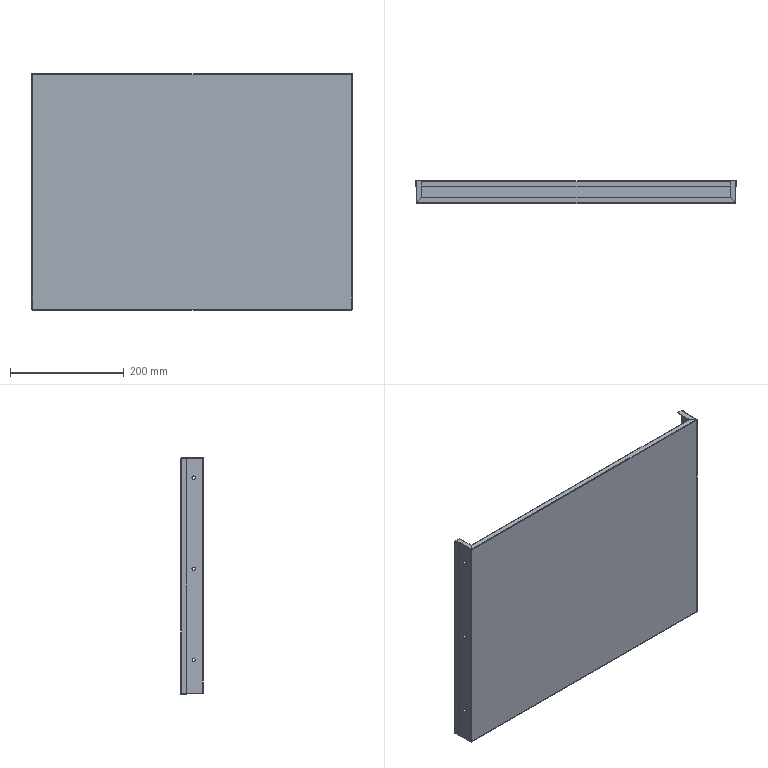Component | SolidWorks | PC-CAJ-P08-1_PC-CAJ-P16-1_PM-CAJ-P56-1 | 1 solid | 99 faces | volume 213582 mm3 | plane 62 | cylinder 33 | spline 4 | commonest cylinder face diameters 6 x12 1 x6 2.4 x6 1.6 x5 0.2 x4 | material Plain Carbon Steel